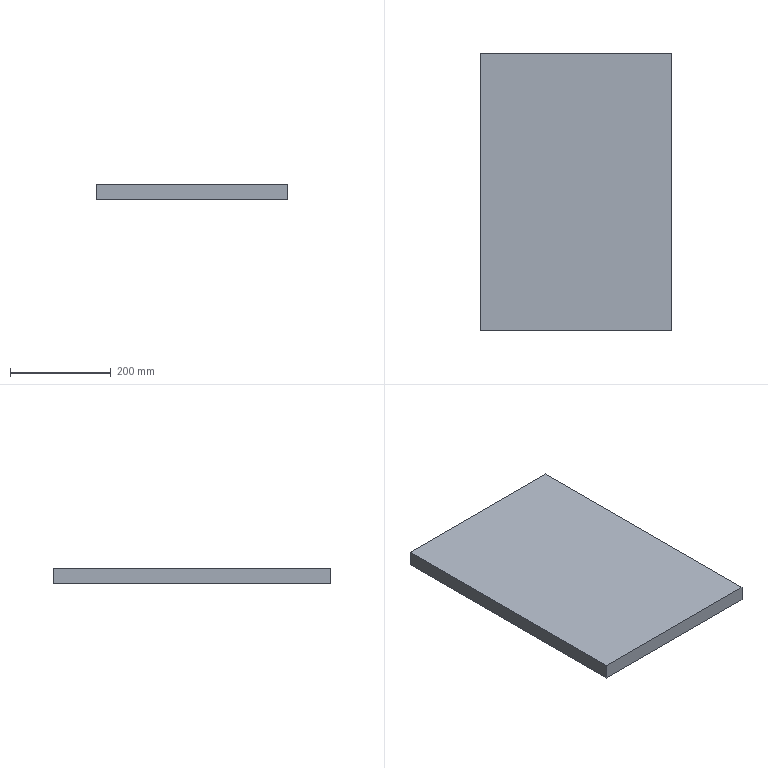Component | SolidWorks | Hanger-1_HangerBasePlate-1 | 1 solid | 6 faces | box 380 x 550 x 30 mm | volume 6270000 mm3 | plane 6 | material Plain Carbon Steel
STEP:
#1=COLOUR_RGB('',0.7922,0.8196,0.9333);
#2=FILL_AREA_STYLE_COLOUR('',#1);
#3=FILL_AREA_STYLE('',(#2));
#4=SURFACE_STYLE_FILL_AREA(#3);
#5=SURFACE_SIDE_STYLE('',(#4));
#6=SURFACE_STYLE_USAGE(.BOTH.,#5);
#7=PRESENTATION_STYLE_ASSIGNMENT((#6));
#8=CARTESIAN_POINT('',(392.698,116.604,265.12));
#9=VERTEX_POINT('',#8);
#10=CARTESIAN_POINT('',(407.659,116.604,265.12));
#11=VERTEX_POINT('',#10);
#12=CARTESIAN_POINT('',(392.698,116.604,265.12));
#13=DIRECTION('',(1.,0.,-0.));
#14=VECTOR('',#13,39.37);
#15=LINE('',#12,#14);
#16=EDGE_CURVE('',#9,#11,#15,.T.);
#17=ORIENTED_EDGE('',*,*,#16,.F.);
#18=CARTESIAN_POINT('',(392.698,116.604,263.939));
#19=VERTEX_POINT('',#18);
#20=CARTESIAN_POINT('',(392.698,116.604,263.939));
#21=DIRECTION('',(0.,0.,1.));
#22=VECTOR('',#21,39.37);
#23=LINE('',#20,#22);
#24=EDGE_CURVE('',#19,#9,#23,.T.);
#25=ORIENTED_EDGE('',*,*,#24,.F.);
#26=CARTESIAN_POINT('',(407.659,116.604,263.939));
#27=VERTEX_POINT('',#26);
#28=CARTESIAN_POINT('',(392.698,116.604,263.939));
#29=DIRECTION('',(1.,0.,-0.));
#30=VECTOR('',#29,39.37);
#31=LINE('',#28,#30);
#32=EDGE_CURVE('',#19,#27,#31,.T.);
#33=ORIENTED_EDGE('',*,*,#32,.T.);
#34=CARTESIAN_POINT('',(407.659,116.604,263.939));
#35=DIRECTION('',(0.,0.,1.));
#36=VECTOR('',#35,39.37);
#37=LINE('',#34,#36);
#38=EDGE_CURVE('',#27,#11,#37,.T.);
#39=ORIENTED_EDGE('',*,*,#38,.T.);
#40=EDGE_LOOP('',(#17,#25,#33,#39));
#41=FACE_OUTER_BOUND('',#40,.T.);
#42=CARTESIAN_POINT('',(392.698,116.604,263.939));
#43=DIRECTION('',(0.,-1.,-0.));
#44=DIRECTION('',(1.,0.,-0.));
#45=AXIS2_PLACEMENT_3D('',#42,#43,#44);
#46=PLANE('',#45);
#47=ADVANCED_FACE('',(#41),#46,.T.);
#48=CARTESIAN_POINT('',(392.698,138.257,265.12));
#49=VERTEX_POINT('',#48);
#50=CARTESIAN_POINT('',(392.698,116.604,265.12));
#51=DIRECTION('',(0.,-1.,0.));
#52=VECTOR('',#51,39.37);
#53=LINE('',#50,#52);
#54=EDGE_CURVE('',#49,#9,#53,.T.);
#55=ORIENTED_EDGE('',*,*,#54,.F.);
#56=CARTESIAN_POINT('',(392.698,138.257,263.939));
#57=VERTEX_POINT('',#56);
#58=CARTESIAN_POINT('',(392.698,138.257,263.939));
#59=DIRECTION('',(0.,0.,1.));
#60=VECTOR('',#59,39.37);
#61=LINE('',#58,#60);
#62=EDGE_CURVE('',#57,#49,#61,.T.);
#63=ORIENTED_EDGE('',*,*,#62,.F.);
#64=CARTESIAN_POINT('',(392.698,116.604,263.939));
#65=DIRECTION('',(0.,-1.,0.));
#66=VECTOR('',#65,39.37);
#67=LINE('',#64,#66);
#68=EDGE_CURVE('',#57,#19,#67,.T.);
#69=ORIENTED_EDGE('',*,*,#68,.T.);
#70=ORIENTED_EDGE('',*,*,#24,.T.);
#71=EDGE_LOOP('',(#55,#63,#69,#70));
#72=FACE_OUTER_BOUND('',#71,.T.);
#73=CARTESIAN_POINT('',(392.698,116.604,263.939));
#74=DIRECTION('',(-1.,-0.,0.));
#75=DIRECTION('',(0.,-1.,0.));
#76=AXIS2_PLACEMENT_3D('',#73,#74,#75);
#77=PLANE('',#76);
#78=ADVANCED_FACE('',(#72),#77,.T.);
#79=CARTESIAN_POINT('',(407.659,138.257,265.12));
#80=VERTEX_POINT('',#79);
#81=CARTESIAN_POINT('',(392.698,138.257,265.12));
#82=DIRECTION('',(-1.,-0.,0.));
#83=VECTOR('',#82,39.37);
#84=LINE('',#81,#83);
#85=EDGE_CURVE('',#80,#49,#84,.T.);
#86=ORIENTED_EDGE('',*,*,#85,.F.);
#87=CARTESIAN_POINT('',(407.659,138.257,263.939));
#88=VERTEX_POINT('',#87);
#89=CARTESIAN_POINT('',(407.659,138.257,263.939));
#90=DIRECTION('',(0.,0.,1.));
#91=VECTOR('',#90,39.37);
#92=LINE('',#89,#91);
#93=EDGE_CURVE('',#88,#80,#92,.T.);
#94=ORIENTED_EDGE('',*,*,#93,.F.);
#95=CARTESIAN_POINT('',(392.698,138.257,263.939));
#96=DIRECTION('',(-1.,-0.,0.));
#97=VECTOR('',#96,39.37);
#98=LINE('',#95,#97);
#99=EDGE_CURVE('',#88,#57,#98,.T.);
#100=ORIENTED_EDGE('',*,*,#99,.T.);
#101=ORIENTED_EDGE('',*,*,#62,.T.);
#102=EDGE_LOOP('',(#86,#94,#100,#101));
#103=FACE_OUTER_BOUND('',#102,.T.);
#104=CARTESIAN_POINT('',(392.698,138.257,263.939));
#105=DIRECTION('',(-0.,1.,-0.));
#106=DIRECTION('',(-1.,-0.,0.));
#107=AXIS2_PLACEMENT_3D('',#104,#105,#106);
#108=PLANE('',#107);
#109=ADVANCED_FACE('',(#103),#108,.T.);
#110=CARTESIAN_POINT('',(407.659,116.604,265.12));
#111=DIRECTION('',(-0.,1.,0.));
#112=VECTOR('',#111,39.37);
#113=LINE('',#110,#112);
#114=EDGE_CURVE('',#11,#80,#113,.T.);
#115=ORIENTED_EDGE('',*,*,#114,.F.);
#116=ORIENTED_EDGE('',*,*,#38,.F.);
#117=CARTESIAN_POINT('',(407.659,116.604,263.939));
#118=DIRECTION('',(-0.,1.,0.));
#119=VECTOR('',#118,39.37);
#120=LINE('',#117,#119);
#121=EDGE_CURVE('',#27,#88,#120,.T.);
#122=ORIENTED_EDGE('',*,*,#121,.T.);
#123=ORIENTED_EDGE('',*,*,#93,.T.);
#124=EDGE_LOOP('',(#115,#116,#122,#123));
#125=FACE_OUTER_BOUND('',#124,.T.);
#126=CARTESIAN_POINT('',(407.659,116.604,263.939));
#127=DIRECTION('',(1.,0.,-0.));
#128=DIRECTION('',(-0.,1.,0.));
#129=AXIS2_PLACEMENT_3D('',#126,#127,#128);
#130=PLANE('',#129);
#131=ADVANCED_FACE('',(#125),#130,.T.);
#132=ORIENTED_EDGE('',*,*,#32,.F.);
#133=ORIENTED_EDGE('',*,*,#68,.F.);
#134=ORIENTED_EDGE('',*,*,#99,.F.);
#135=ORIENTED_EDGE('',*,*,#121,.F.);
#136=EDGE_LOOP('',(#132,#133,#134,#135));
#137=FACE_OUTER_BOUND('',#136,.T.);
#138=CARTESIAN_POINT('',(392.698,116.604,263.939));
#139=DIRECTION('',(0.,0.,1.));
#140=DIRECTION('',(1.,0.,-0.));
#141=AXIS2_PLACEMENT_3D('',#138,#139,#140);
#142=PLANE('',#141);
#143=ADVANCED_FACE('',(#137),#142,.F.);
#144=ORIENTED_EDGE('',*,*,#16,.T.);
#145=ORIENTED_EDGE('',*,*,#114,.T.);
#146=ORIENTED_EDGE('',*,*,#85,.T.);
#147=ORIENTED_EDGE('',*,*,#54,.T.);
#148=EDGE_LOOP('',(#144,#145,#146,#147));
#149=FACE_OUTER_BOUND('',#148,.T.);
#150=CARTESIAN_POINT('',(392.698,116.604,265.12));
#151=DIRECTION('',(0.,0.,1.));
#152=DIRECTION('',(1.,0.,-0.));
#153=AXIS2_PLACEMENT_3D('',#150,#151,#152);
#154=PLANE('',#153);
#155=ADVANCED_FACE('',(#149),#154,.T.);
#156=CLOSED_SHELL('',(#47,#78,#109,#131,#143,#155));
#157=MANIFOLD_SOLID_BREP('',#156);
#158=STYLED_ITEM('',(#7),#157);
#159=PRESENTATION_LAYER_ASSIGNMENT('','',(#158));
#160=CARTESIAN_POINT('',(0.,0.,0.));
#161=DIRECTION('',(0.,0.,1.));
#162=DIRECTION('',(1.,0.,0.));
#163=AXIS2_PLACEMENT_3D('',#160,#161,#162);
#164=(LENGTH_UNIT()NAMED_UNIT(*)SI_UNIT($,.METRE.));
#165=LENGTH_MEASURE_WITH_UNIT(LENGTH_MEASURE(0.0254),#164);
#166=DIMENSIONAL_EXPONENTS(1.,0.,0.,0.,0.,0.,0.);
#167=(CONVERSION_BASED_UNIT('',#165)LENGTH_UNIT()NAMED_UNIT(#166));
#168=UNCERTAINTY_MEASURE_WITH_UNIT(LENGTH_MEASURE(0.00001),#167,'','');
#169=(NAMED_UNIT(*)PLANE_ANGLE_UNIT()SI_UNIT($,.RADIAN.));
#170=(NAMED_UNIT(*)SI_UNIT($,.STERADIAN.)SOLID_ANGLE_UNIT());
#171=(GEOMETRIC_REPRESENTATION_CONTEXT(3)GLOBAL_UNCERTAINTY_ASSIGNED_CONTEXT((#168))GLOBAL_UNIT_ASSIGNED_CONTEXT((#167,#169,#170))REPRESENTATION_CONTEXT('',''));
#172=ADVANCED_BREP_SHAPE_REPRESENTATION('',(#157,#163),#171);
#173=(LENGTH_UNIT()NAMED_UNIT(*)SI_UNIT($,.METRE.));
#174=LENGTH_MEASURE_WITH_UNIT(LENGTH_MEASURE(0.0254),#173);
#175=DIMENSIONAL_EXPONENTS(1.,0.,0.,0.,0.,0.,0.);
#176=(CONVERSION_BASED_UNIT('',#174)LENGTH_UNIT()NAMED_UNIT(#175));
#177=UNCERTAINTY_MEASURE_WITH_UNIT(LENGTH_MEASURE(0.00001),#176,'','');
#178=(NAMED_UNIT(*)PLANE_ANGLE_UNIT()SI_UNIT($,.RADIAN.));
#179=(NAMED_UNIT(*)SI_UNIT($,.STERADIAN.)SOLID_ANGLE_UNIT());
#180=(GEOMETRIC_REPRESENTATION_CONTEXT(3)GLOBAL_UNCERTAINTY_ASSIGNED_CONTEXT((#177))GLOBAL_UNIT_ASSIGNED_CONTEXT((#176,#178,#179))REPRESENTATION_CONTEXT('',''));
#181=MECHANICAL_DESIGN_GEOMETRIC_PRESENTATION_REPRESENTATION('',(#158),#180);